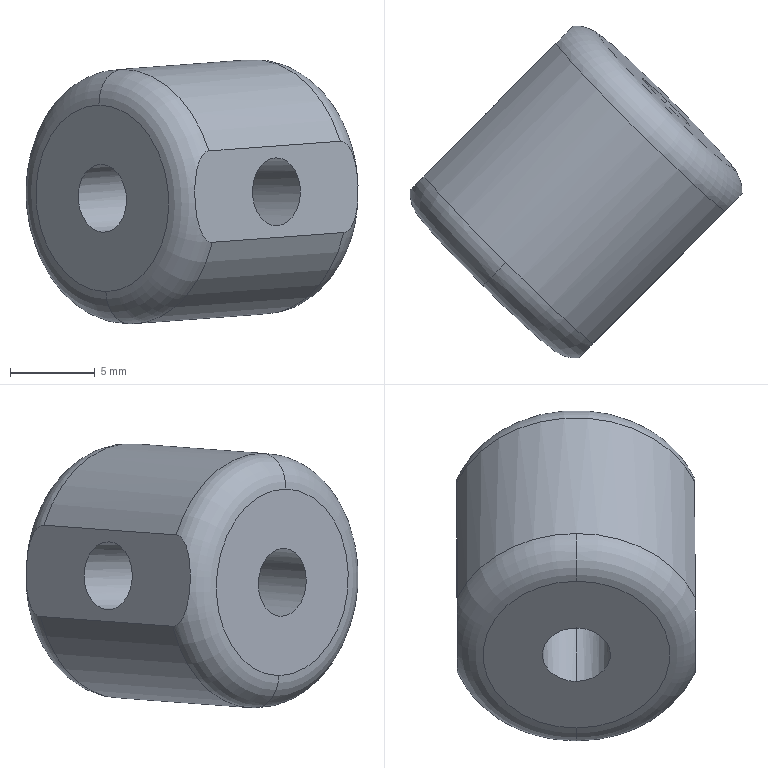Component | SolidWorks | DoubleFilmTransport-1_CrossJoint-3 | 1 solid | 19 faces | box 19.56 x 19.56 x 15.56 mm | volume 2207 mm3 | cylinder 11 | torus 4 | plane 4 | commonest cylinder face diameters 4 x8 15 x3
STEP:
#1=COLOUR_RGB('',0.7922,0.8196,0.9333);
#2=FILL_AREA_STYLE_COLOUR('',#1);
#3=FILL_AREA_STYLE('',(#2));
#4=SURFACE_STYLE_FILL_AREA(#3);
#5=SURFACE_SIDE_STYLE('',(#4));
#6=SURFACE_STYLE_USAGE(.BOTH.,#5);
#7=PRESENTATION_STYLE_ASSIGNMENT((#6));
#8=CARTESIAN_POINT('',(-15.09,3.644,-2.839));
#9=VERTEX_POINT('',#8);
#10=CARTESIAN_POINT('',(-14.783,3.339,-2.839));
#11=VERTEX_POINT('',#10);
#12=CARTESIAN_POINT('',(-14.937,3.492,-2.839));
#13=DIRECTION('',(-0.704,-0.7083,-0.05198));
#14=DIRECTION('',(-0.7092,0.705,0.));
#15=AXIS2_PLACEMENT_3D('',#12,#13,#14);
#16=CIRCLE('',#15,0.2165);
#17=EDGE_CURVE('',#9,#11,#16,.T.);
#18=ORIENTED_EDGE('',*,*,#17,.T.);
#19=CARTESIAN_POINT('',(-14.76,3.278,-2.84));
#20=VERTEX_POINT('',#19);
#21=CARTESIAN_POINT('',(-14.839,3.283,-2.843));
#22=DIRECTION('',(0.03664,0.03687,-0.9986));
#23=DIRECTION('',(0.,0.9993,0.03689));
#24=AXIS2_PLACEMENT_3D('',#21,#22,#23);
#25=CIRCLE('',#24,0.07874);
#26=EDGE_CURVE('',#11,#20,#25,.T.);
#27=ORIENTED_EDGE('',*,*,#26,.T.);
#28=CARTESIAN_POINT('',(-14.793,3.245,-2.949));
#29=VERTEX_POINT('',#28);
#30=CARTESIAN_POINT('',(-14.76,3.278,-2.84));
#31=CARTESIAN_POINT('',(-14.76,3.279,-2.851));
#32=CARTESIAN_POINT('',(-14.76,3.279,-2.862));
#33=CARTESIAN_POINT('',(-14.761,3.277,-2.883));
#34=CARTESIAN_POINT('',(-14.762,3.276,-2.893));
#35=CARTESIAN_POINT('',(-14.767,3.272,-2.914));
#36=CARTESIAN_POINT('',(-14.77,3.269,-2.924));
#37=CARTESIAN_POINT('',(-14.776,3.262,-2.937));
#38=CARTESIAN_POINT('',(-14.779,3.259,-2.941));
#39=CARTESIAN_POINT('',(-14.784,3.255,-2.945));
#40=CARTESIAN_POINT('',(-14.786,3.253,-2.947));
#41=CARTESIAN_POINT('',(-14.789,3.249,-2.948));
#42=CARTESIAN_POINT('',(-14.791,3.247,-2.949));
#43=CARTESIAN_POINT('',(-14.793,3.245,-2.949));
#44=B_SPLINE_CURVE_WITH_KNOTS('',3,(#30,#31,#32,#33,#34,#35,#36,#37,#38,#39,#40,#41,#42,#43),.UNSPECIFIED.,.F.,.F.,(4,2,2,2,2,2,4),(0.00327,0.004088,0.004906,0.005724,0.006133,0.006337,0.006542),.UNSPECIFIED.);
#45=EDGE_CURVE('',#20,#29,#44,.T.);
#46=ORIENTED_EDGE('',*,*,#45,.T.);
#47=CARTESIAN_POINT('',(-14.981,3.447,-3.138));
#48=VERTEX_POINT('',#47);
#49=CARTESIAN_POINT('',(-14.992,3.436,-2.843));
#50=DIRECTION('',(0.704,0.7083,0.05198));
#51=DIRECTION('',(-0.03664,-0.03687,0.9986));
#52=AXIS2_PLACEMENT_3D('',#49,#50,#51);
#53=CIRCLE('',#52,0.2953);
#54=EDGE_CURVE('',#29,#48,#53,.T.);
#55=ORIENTED_EDGE('',*,*,#54,.T.);
#56=CARTESIAN_POINT('',(-15.184,3.634,-2.949));
#57=VERTEX_POINT('',#56);
#58=CARTESIAN_POINT('',(-14.992,3.436,-2.843));
#59=DIRECTION('',(0.704,0.7083,0.05198));
#60=DIRECTION('',(-0.03664,-0.03687,0.9986));
#61=AXIS2_PLACEMENT_3D('',#58,#59,#60);
#62=CIRCLE('',#61,0.2953);
#63=EDGE_CURVE('',#48,#57,#62,.T.);
#64=ORIENTED_EDGE('',*,*,#63,.T.);
#65=CARTESIAN_POINT('',(-15.151,3.667,-2.84));
#66=VERTEX_POINT('',#65);
#67=CARTESIAN_POINT('',(-15.184,3.634,-2.949));
#68=CARTESIAN_POINT('',(-15.18,3.638,-2.949));
#69=CARTESIAN_POINT('',(-15.176,3.642,-2.947));
#70=CARTESIAN_POINT('',(-15.17,3.648,-2.941));
#71=CARTESIAN_POINT('',(-15.167,3.651,-2.937));
#72=CARTESIAN_POINT('',(-15.163,3.655,-2.928));
#73=CARTESIAN_POINT('',(-15.161,3.657,-2.924));
#74=CARTESIAN_POINT('',(-15.158,3.66,-2.914));
#75=CARTESIAN_POINT('',(-15.156,3.662,-2.909));
#76=CARTESIAN_POINT('',(-15.153,3.665,-2.893));
#77=CARTESIAN_POINT('',(-15.152,3.666,-2.883));
#78=CARTESIAN_POINT('',(-15.151,3.667,-2.862));
#79=CARTESIAN_POINT('',(-15.151,3.667,-2.851));
#80=CARTESIAN_POINT('',(-15.151,3.667,-2.84));
#81=B_SPLINE_CURVE_WITH_KNOTS('',3,(#67,#68,#69,#70,#71,#72,#73,#74,#75,#76,#77,#78,#79,#80),.UNSPECIFIED.,.F.,.F.,(4,2,2,2,2,2,4),(0.,0.0004087,0.0008174,0.001226,0.001635,0.002452,0.00327),.UNSPECIFIED.);
#82=EDGE_CURVE('',#57,#66,#81,.T.);
#83=ORIENTED_EDGE('',*,*,#82,.T.);
#84=CARTESIAN_POINT('',(-15.146,3.588,-2.843));
#85=DIRECTION('',(-0.03664,-0.03687,0.9986));
#86=DIRECTION('',(0.,-0.9993,-0.03689));
#87=AXIS2_PLACEMENT_3D('',#84,#85,#86);
#88=CIRCLE('',#87,0.07874);
#89=EDGE_CURVE('',#9,#66,#88,.T.);
#90=ORIENTED_EDGE('',*,*,#89,.F.);
#91=EDGE_LOOP('',(#18,#27,#46,#55,#64,#83,#90));
#92=FACE_OUTER_BOUND('',#91,.T.);
#93=CARTESIAN_POINT('',(-14.992,3.436,-2.843));
#94=DIRECTION('',(-0.704,-0.7083,-0.05198));
#95=DIRECTION('',(-0.7092,0.705,0.));
#96=AXIS2_PLACEMENT_3D('',#93,#94,#95);
#97=TOROIDAL_SURFACE('',#96,0.2165,0.07874);
#98=ADVANCED_FACE('',(#92),#97,.T.);
#99=CARTESIAN_POINT('',(-15.308,3.118,-2.571));
#100=VERTEX_POINT('',#99);
#101=CARTESIAN_POINT('',(-15.106,2.931,-2.76));
#102=VERTEX_POINT('',#101);
#103=CARTESIAN_POINT('',(-15.297,3.129,-2.866));
#104=DIRECTION('',(0.704,0.7083,0.05198));
#105=DIRECTION('',(0.03664,0.03687,-0.9986));
#106=AXIS2_PLACEMENT_3D('',#103,#104,#105);
#107=CIRCLE('',#106,0.2953);
#108=EDGE_CURVE('',#100,#102,#107,.T.);
#109=ORIENTED_EDGE('',*,*,#108,.F.);
#110=CARTESIAN_POINT('',(-15.361,3.065,-2.653));
#111=VERTEX_POINT('',#110);
#112=CARTESIAN_POINT('',(-15.305,3.121,-2.649));
#113=DIRECTION('',(0.7092,-0.705,0.));
#114=DIRECTION('',(0.705,0.7092,0.));
#115=AXIS2_PLACEMENT_3D('',#112,#113,#114);
#116=CIRCLE('',#115,0.07874);
#117=EDGE_CURVE('',#100,#111,#116,.T.);
#118=ORIENTED_EDGE('',*,*,#117,.T.);
#119=CARTESIAN_POINT('',(-15.345,3.081,-3.086));
#120=VERTEX_POINT('',#119);
#121=CARTESIAN_POINT('',(-15.353,3.073,-2.87));
#122=DIRECTION('',(0.704,0.7083,0.05198));
#123=DIRECTION('',(0.03664,0.03687,-0.9986));
#124=AXIS2_PLACEMENT_3D('',#121,#122,#123);
#125=CIRCLE('',#124,0.2165);
#126=EDGE_CURVE('',#111,#120,#125,.T.);
#127=ORIENTED_EDGE('',*,*,#126,.T.);
#128=CARTESIAN_POINT('',(-15.286,3.14,-3.16));
#129=VERTEX_POINT('',#128);
#130=CARTESIAN_POINT('',(-15.289,3.137,-3.082));
#131=DIRECTION('',(-0.7092,0.705,-0.));
#132=DIRECTION('',(-0.705,-0.7092,0.));
#133=AXIS2_PLACEMENT_3D('',#130,#131,#132);
#134=CIRCLE('',#133,0.07874);
#135=EDGE_CURVE('',#129,#120,#134,.T.);
#136=ORIENTED_EDGE('',*,*,#135,.F.);
#137=CARTESIAN_POINT('',(-15.098,2.939,-2.971));
#138=VERTEX_POINT('',#137);
#139=CARTESIAN_POINT('',(-15.297,3.129,-2.866));
#140=DIRECTION('',(-0.704,-0.7083,-0.05198));
#141=DIRECTION('',(0.03664,0.03687,-0.9986));
#142=AXIS2_PLACEMENT_3D('',#139,#140,#141);
#143=CIRCLE('',#142,0.2953);
#144=EDGE_CURVE('',#129,#138,#143,.T.);
#145=ORIENTED_EDGE('',*,*,#144,.T.);
#146=CARTESIAN_POINT('',(-15.098,2.939,-2.971));
#147=CARTESIAN_POINT('',(-15.102,2.935,-2.972));
#148=CARTESIAN_POINT('',(-15.105,2.931,-2.97));
#149=CARTESIAN_POINT('',(-15.112,2.924,-2.965));
#150=CARTESIAN_POINT('',(-15.115,2.921,-2.962));
#151=CARTESIAN_POINT('',(-15.12,2.916,-2.954));
#152=CARTESIAN_POINT('',(-15.123,2.914,-2.95));
#153=CARTESIAN_POINT('',(-15.126,2.91,-2.941));
#154=CARTESIAN_POINT('',(-15.128,2.908,-2.936));
#155=CARTESIAN_POINT('',(-15.132,2.904,-2.921));
#156=CARTESIAN_POINT('',(-15.134,2.902,-2.91));
#157=CARTESIAN_POINT('',(-15.137,2.899,-2.89));
#158=CARTESIAN_POINT('',(-15.138,2.898,-2.879));
#159=CARTESIAN_POINT('',(-15.139,2.897,-2.858));
#160=CARTESIAN_POINT('',(-15.139,2.898,-2.847));
#161=CARTESIAN_POINT('',(-15.137,2.899,-2.826));
#162=CARTESIAN_POINT('',(-15.136,2.9,-2.815));
#163=CARTESIAN_POINT('',(-15.132,2.904,-2.795));
#164=CARTESIAN_POINT('',(-15.129,2.907,-2.784));
#165=CARTESIAN_POINT('',(-15.122,2.914,-2.772));
#166=CARTESIAN_POINT('',(-15.119,2.917,-2.768));
#167=CARTESIAN_POINT('',(-15.113,2.923,-2.762));
#168=CARTESIAN_POINT('',(-15.109,2.927,-2.76));
#169=CARTESIAN_POINT('',(-15.106,2.931,-2.76));
#170=B_SPLINE_CURVE_WITH_KNOTS('',3,(#146,#147,#148,#149,#150,#151,#152,#153,#154,#155,#156,#157,#158,#159,#160,#161,#162,#163,#164,#165,#166,#167,#168,#169),.UNSPECIFIED.,.F.,.F.,(4,2,2,2,2,2,2,2,2,2,2,4),(0.,0.0004088,0.0008177,0.001227,0.001635,0.002453,0.003271,0.004088,0.004906,0.005724,0.006133,0.006542),.UNSPECIFIED.);
#171=EDGE_CURVE('',#138,#102,#170,.T.);
#172=ORIENTED_EDGE('',*,*,#171,.T.);
#173=EDGE_LOOP('',(#109,#118,#127,#136,#145,#172));
#174=FACE_OUTER_BOUND('',#173,.T.);
#175=CARTESIAN_POINT('',(-15.297,3.129,-2.866));
#176=DIRECTION('',(-0.704,-0.7083,-0.05198));
#177=DIRECTION('',(0.03664,0.03687,-0.9986));
#178=AXIS2_PLACEMENT_3D('',#175,#176,#177);
#179=TOROIDAL_SURFACE('',#178,0.2165,0.07874);
#180=ADVANCED_FACE('',(#174),#179,.T.);
#181=CARTESIAN_POINT('',(-15.337,3.48,-2.933));
#182=VERTEX_POINT('',#181);
#183=CARTESIAN_POINT('',(-15.343,3.474,-2.776));
#184=VERTEX_POINT('',#183);
#185=CARTESIAN_POINT('',(-15.34,3.477,-2.854));
#186=DIRECTION('',(-0.7092,0.705,-0.));
#187=DIRECTION('',(0.03664,0.03687,-0.9986));
#188=AXIS2_PLACEMENT_3D('',#185,#186,#187);
#189=CIRCLE('',#188,0.07874);
#190=EDGE_CURVE('',#182,#184,#189,.T.);
#191=ORIENTED_EDGE('',*,*,#190,.T.);
#192=CARTESIAN_POINT('',(-15.148,3.28,-2.776));
#193=VERTEX_POINT('',#192);
#194=CARTESIAN_POINT('',(-15.343,3.474,-2.776));
#195=DIRECTION('',(0.7092,-0.705,0.));
#196=VECTOR('',#195,39.37);
#197=LINE('',#194,#196);
#198=EDGE_CURVE('',#184,#193,#197,.T.);
#199=ORIENTED_EDGE('',*,*,#198,.T.);
#200=CARTESIAN_POINT('',(-15.142,3.285,-2.933));
#201=VERTEX_POINT('',#200);
#202=CARTESIAN_POINT('',(-15.142,3.285,-2.933));
#203=CARTESIAN_POINT('',(-15.364,3.285,-2.941));
#204=CARTESIAN_POINT('',(-15.37,3.279,-2.784));
#205=CARTESIAN_POINT('',(-15.148,3.28,-2.776));
#206=(BOUNDED_CURVE()B_SPLINE_CURVE(3,(#202,#203,#204,#205),.UNSPECIFIED.,.F.,.T.)B_SPLINE_CURVE_WITH_KNOTS((4,4),(4.712,7.854),.UNSPECIFIED.)CURVE()GEOMETRIC_REPRESENTATION_ITEM()RATIONAL_B_SPLINE_CURVE((1.,0.3333,0.3333,1.))REPRESENTATION_ITEM(''));
#207=EDGE_CURVE('',#201,#193,#206,.T.);
#208=ORIENTED_EDGE('',*,*,#207,.F.);
#209=CARTESIAN_POINT('',(-15.337,3.48,-2.933));
#210=DIRECTION('',(0.7092,-0.705,0.));
#211=VECTOR('',#210,39.37);
#212=LINE('',#209,#211);
#213=EDGE_CURVE('',#182,#201,#212,.T.);
#214=ORIENTED_EDGE('',*,*,#213,.F.);
#215=EDGE_LOOP('',(#191,#199,#208,#214));
#216=FACE_OUTER_BOUND('',#215,.T.);
#217=CARTESIAN_POINT('',(-15.34,3.477,-2.854));
#218=DIRECTION('',(0.7092,-0.705,0.));
#219=DIRECTION('',(0.03664,0.03687,-0.9986));
#220=AXIS2_PLACEMENT_3D('',#217,#218,#219);
#221=CYLINDRICAL_SURFACE('',#220,0.07874);
#222=ADVANCED_FACE('',(#216),#221,.F.);
#223=ORIENTED_EDGE('',*,*,#63,.F.);
#224=CARTESIAN_POINT('',(-15.296,3.13,-3.161));
#225=DIRECTION('',(-0.704,-0.7083,-0.05198));
#226=VECTOR('',#225,39.37);
#227=LINE('',#224,#226);
#228=EDGE_CURVE('',#48,#129,#227,.T.);
#229=ORIENTED_EDGE('',*,*,#228,.T.);
#230=CARTESIAN_POINT('',(-15.489,3.327,-2.971));
#231=VERTEX_POINT('',#230);
#232=CARTESIAN_POINT('',(-15.297,3.129,-2.866));
#233=DIRECTION('',(-0.704,-0.7083,-0.05198));
#234=DIRECTION('',(0.03664,0.03687,-0.9986));
#235=AXIS2_PLACEMENT_3D('',#232,#233,#234);
#236=CIRCLE('',#235,0.2953);
#237=EDGE_CURVE('',#231,#129,#236,.T.);
#238=ORIENTED_EDGE('',*,*,#237,.F.);
#239=CARTESIAN_POINT('',(-15.128,3.69,-2.945));
#240=DIRECTION('',(0.704,0.7083,0.05198));
#241=VECTOR('',#240,39.37);
#242=LINE('',#239,#241);
#243=EDGE_CURVE('',#231,#57,#242,.T.);
#244=ORIENTED_EDGE('',*,*,#243,.T.);
#245=EDGE_LOOP('',(#223,#229,#238,#244));
#246=FACE_OUTER_BOUND('',#245,.T.);
#247=CARTESIAN_POINT('',(-15.307,3.119,-2.866));
#248=DIRECTION('',(-0.704,-0.7083,-0.05198));
#249=DIRECTION('',(0.03664,0.03687,-0.9986));
#250=AXIS2_PLACEMENT_3D('',#247,#248,#249);
#251=CYLINDRICAL_SURFACE('',#250,0.2953);
#252=ADVANCED_FACE('',(#246),#251,.T.);
#253=CARTESIAN_POINT('',(-15.148,3.28,-2.776));
#254=CARTESIAN_POINT('',(-15.148,3.273,-2.776));
#255=CARTESIAN_POINT('',(-15.148,3.266,-2.777));
#256=CARTESIAN_POINT('',(-15.148,3.259,-2.778));
#257=CARTESIAN_POINT('',(-15.147,3.256,-2.778));
#258=CARTESIAN_POINT('',(-15.147,3.253,-2.779));
#259=CARTESIAN_POINT('',(-15.147,3.252,-2.779));
#260=CARTESIAN_POINT('',(-15.147,3.25,-2.78));
#261=CARTESIAN_POINT('',(-15.147,3.249,-2.78));
#262=CARTESIAN_POINT('',(-15.147,3.249,-2.78));
#263=CARTESIAN_POINT('',(-15.147,3.249,-2.78));
#264=CARTESIAN_POINT('',(-15.147,3.249,-2.78));
#265=CARTESIAN_POINT('',(-15.147,3.249,-2.78));
#266=CARTESIAN_POINT('',(-15.147,3.241,-2.782));
#267=CARTESIAN_POINT('',(-15.147,3.235,-2.784));
#268=CARTESIAN_POINT('',(-15.147,3.226,-2.787));
#269=CARTESIAN_POINT('',(-15.147,3.223,-2.789));
#270=CARTESIAN_POINT('',(-15.147,3.219,-2.791));
#271=CARTESIAN_POINT('',(-15.147,3.217,-2.792));
#272=CARTESIAN_POINT('',(-15.147,3.215,-2.793));
#273=CARTESIAN_POINT('',(-15.147,3.214,-2.793));
#274=CARTESIAN_POINT('',(-15.147,3.214,-2.794));
#275=CARTESIAN_POINT('',(-15.147,3.214,-2.794));
#276=CARTESIAN_POINT('',(-15.147,3.214,-2.794));
#277=CARTESIAN_POINT('',(-15.147,3.207,-2.798));
#278=CARTESIAN_POINT('',(-15.146,3.201,-2.802));
#279=CARTESIAN_POINT('',(-15.146,3.193,-2.809));
#280=CARTESIAN_POINT('',(-15.146,3.191,-2.811));
#281=CARTESIAN_POINT('',(-15.146,3.188,-2.815));
#282=CARTESIAN_POINT('',(-15.146,3.186,-2.817));
#283=CARTESIAN_POINT('',(-15.146,3.184,-2.819));
#284=CARTESIAN_POINT('',(-15.146,3.184,-2.82));
#285=CARTESIAN_POINT('',(-15.146,3.183,-2.82));
#286=CARTESIAN_POINT('',(-15.146,3.183,-2.821));
#287=CARTESIAN_POINT('',(-15.145,3.175,-2.833));
#288=CARTESIAN_POINT('',(-15.145,3.171,-2.846));
#289=CARTESIAN_POINT('',(-15.144,3.171,-2.865));
#290=CARTESIAN_POINT('',(-15.144,3.173,-2.871));
#291=CARTESIAN_POINT('',(-15.144,3.176,-2.88));
#292=CARTESIAN_POINT('',(-15.143,3.178,-2.883));
#293=CARTESIAN_POINT('',(-15.143,3.18,-2.888));
#294=CARTESIAN_POINT('',(-15.143,3.182,-2.89));
#295=CARTESIAN_POINT('',(-15.143,3.184,-2.892));
#296=CARTESIAN_POINT('',(-15.143,3.184,-2.894));
#297=CARTESIAN_POINT('',(-15.143,3.185,-2.894));
#298=CARTESIAN_POINT('',(-15.143,3.185,-2.895));
#299=CARTESIAN_POINT('',(-15.143,3.189,-2.9));
#300=CARTESIAN_POINT('',(-15.143,3.194,-2.904));
#301=CARTESIAN_POINT('',(-15.143,3.202,-2.91));
#302=CARTESIAN_POINT('',(-15.142,3.205,-2.912));
#303=CARTESIAN_POINT('',(-15.142,3.21,-2.915));
#304=CARTESIAN_POINT('',(-15.142,3.212,-2.917));
#305=CARTESIAN_POINT('',(-15.142,3.215,-2.918));
#306=CARTESIAN_POINT('',(-15.142,3.216,-2.919));
#307=CARTESIAN_POINT('',(-15.142,3.217,-2.919));
#308=CARTESIAN_POINT('',(-15.142,3.218,-2.919));
#309=CARTESIAN_POINT('',(-15.142,3.218,-2.92));
#310=CARTESIAN_POINT('',(-15.142,3.223,-2.922));
#311=CARTESIAN_POINT('',(-15.142,3.228,-2.924));
#312=CARTESIAN_POINT('',(-15.142,3.237,-2.927));
#313=CARTESIAN_POINT('',(-15.142,3.24,-2.928));
#314=CARTESIAN_POINT('',(-15.142,3.245,-2.929));
#315=CARTESIAN_POINT('',(-15.142,3.248,-2.93));
#316=CARTESIAN_POINT('',(-15.142,3.251,-2.93));
#317=CARTESIAN_POINT('',(-15.142,3.252,-2.931));
#318=CARTESIAN_POINT('',(-15.142,3.253,-2.931));
#319=CARTESIAN_POINT('',(-15.142,3.254,-2.931));
#320=CARTESIAN_POINT('',(-15.142,3.254,-2.931));
#321=CARTESIAN_POINT('',(-15.142,3.254,-2.931));
#322=CARTESIAN_POINT('',(-15.142,3.261,-2.932));
#323=CARTESIAN_POINT('',(-15.142,3.271,-2.933));
#324=CARTESIAN_POINT('',(-15.142,3.285,-2.933));
#325=B_SPLINE_CURVE_WITH_KNOTS('',3,(#253,#254,#255,#256,#257,#258,#259,#260,#261,#262,#263,#264,#265,#266,#267,#268,#269,#270,#271,#272,#273,#274,#275,#276,#277,#278,#279,#280,#281,#282,#283,#284,#285,#286,#287,#288,#289,#290,#291,#292,#293,#294,#295,#296,#297,#298,#299,#300,#301,#302,#303,#304,#305,#306,#307,#308,#309,#310,#311,#312,#313,#314,#315,#316,#317,#318,#319,#320,#321,#322,#323,#324),.UNSPECIFIED.,.F.,.F.,(4,2,2,1,1,1,1,2,2,2,2,1,1,1,2,2,2,2,1,1,2,2,2,2,2,1,1,2,2,2,2,1,1,1,2,2,2,2,1,1,1,1,2,2,4),(0.,0.0625,0.09375,0.1094,0.1172,0.1211,0.123,0.124,0.125,0.1875,0.2188,0.2344,0.2422,0.2461,0.248,0.25,0.3125,0.3438,0.3594,0.3672,0.3711,0.375,0.5,0.5625,0.5938,0.6094,0.6172,0.6211,0.625,0.6875,0.7188,0.7344,0.7422,0.7461,0.748,0.75,0.8125,0.8438,0.8594,0.8672,0.8711,0.873,0.874,0.875,1.),.UNSPECIFIED.);
#326=EDGE_CURVE('',#193,#201,#325,.T.);
#327=ORIENTED_EDGE('',*,*,#326,.F.);
#328=CARTESIAN_POINT('',(-14.952,3.085,-2.776));
#329=VERTEX_POINT('',#328);
#330=CARTESIAN_POINT('',(-15.343,3.474,-2.776));
#331=DIRECTION('',(0.7092,-0.705,0.));
#332=VECTOR('',#331,39.37);
#333=LINE('',#330,#332);
#334=EDGE_CURVE('',#193,#329,#333,.T.);
#335=ORIENTED_EDGE('',*,*,#334,.T.);
#336=CARTESIAN_POINT('',(-14.946,3.091,-2.933));
#337=VERTEX_POINT('',#336);
#338=CARTESIAN_POINT('',(-14.949,3.088,-2.854));
#339=DIRECTION('',(0.7092,-0.705,0.));
#340=DIRECTION('',(0.03664,0.03687,-0.9986));
#341=AXIS2_PLACEMENT_3D('',#338,#339,#340);
#342=CIRCLE('',#341,0.07874);
#343=EDGE_CURVE('',#329,#337,#342,.T.);
#344=ORIENTED_EDGE('',*,*,#343,.T.);
#345=CARTESIAN_POINT('',(-15.337,3.48,-2.933));
#346=DIRECTION('',(0.7092,-0.705,0.));
#347=VECTOR('',#346,39.37);
#348=LINE('',#345,#347);
#349=EDGE_CURVE('',#201,#337,#348,.T.);
#350=ORIENTED_EDGE('',*,*,#349,.F.);
#351=EDGE_LOOP('',(#327,#335,#344,#350));
#352=FACE_OUTER_BOUND('',#351,.T.);
#353=CARTESIAN_POINT('',(-15.34,3.477,-2.854));
#354=DIRECTION('',(0.7092,-0.705,0.));
#355=DIRECTION('',(0.03664,0.03687,-0.9986));
#356=AXIS2_PLACEMENT_3D('',#353,#354,#355);
#357=CYLINDRICAL_SURFACE('',#356,0.07874);
#358=ADVANCED_FACE('',(#352),#357,.F.);
#359=ORIENTED_EDGE('',*,*,#207,.T.);
#360=CARTESIAN_POINT('',(-15.356,3.07,-2.791));
#361=VERTEX_POINT('',#360);
#362=CARTESIAN_POINT('',(-15.31,3.116,-2.788));
#363=DIRECTION('',(-0.704,-0.7083,-0.05198));
#364=VECTOR('',#363,39.37);
#365=LINE('',#362,#364);
#366=EDGE_CURVE('',#193,#361,#365,.T.);
#367=ORIENTED_EDGE('',*,*,#366,.T.);
#368=CARTESIAN_POINT('',(-15.35,3.076,-2.948));
#369=VERTEX_POINT('',#368);
#370=CARTESIAN_POINT('',(-15.356,3.07,-2.791));
#371=CARTESIAN_POINT('',(-15.363,3.078,-2.791));
#372=CARTESIAN_POINT('',(-15.37,3.085,-2.793));
#373=CARTESIAN_POINT('',(-15.383,3.099,-2.801));
#374=CARTESIAN_POINT('',(-15.389,3.105,-2.807));
#375=CARTESIAN_POINT('',(-15.399,3.116,-2.821));
#376=CARTESIAN_POINT('',(-15.403,3.12,-2.83));
#377=CARTESIAN_POINT('',(-15.408,3.127,-2.849));
#378=CARTESIAN_POINT('',(-15.409,3.128,-2.859));
#379=CARTESIAN_POINT('',(-15.408,3.129,-2.88));
#380=CARTESIAN_POINT('',(-15.406,3.128,-2.89));
#381=CARTESIAN_POINT('',(-15.4,3.123,-2.909));
#382=CARTESIAN_POINT('',(-15.396,3.119,-2.918));
#383=CARTESIAN_POINT('',(-15.385,3.11,-2.933));
#384=CARTESIAN_POINT('',(-15.378,3.104,-2.938));
#385=CARTESIAN_POINT('',(-15.364,3.091,-2.946));
#386=CARTESIAN_POINT('',(-15.357,3.083,-2.948));
#387=CARTESIAN_POINT('',(-15.35,3.076,-2.948));
#388=B_SPLINE_CURVE_WITH_KNOTS('',3,(#370,#371,#372,#373,#374,#375,#376,#377,#378,#379,#380,#381,#382,#383,#384,#385,#386,#387),.UNSPECIFIED.,.F.,.F.,(4,2,2,2,2,2,2,2,4),(0.,0.125,0.25,0.375,0.5,0.625,0.75,0.875,1.),.UNSPECIFIED.);
#389=EDGE_CURVE('',#361,#369,#388,.T.);
#390=ORIENTED_EDGE('',*,*,#389,.T.);
#391=CARTESIAN_POINT('',(-15.304,3.122,-2.945));
#392=DIRECTION('',(-0.704,-0.7083,-0.05198));
#393=VECTOR('',#392,39.37);
#394=LINE('',#391,#393);
#395=EDGE_CURVE('',#201,#369,#394,.T.);
#396=ORIENTED_EDGE('',*,*,#395,.F.);
#397=EDGE_LOOP('',(#359,#367,#390,#396));
#398=FACE_OUTER_BOUND('',#397,.T.);
#399=CARTESIAN_POINT('',(-15.307,3.119,-2.866));
#400=DIRECTION('',(-0.704,-0.7083,-0.05198));
#401=DIRECTION('',(0.03664,0.03687,-0.9986));
#402=AXIS2_PLACEMENT_3D('',#399,#400,#401);
#403=CYLINDRICAL_SURFACE('',#402,0.07874);
#404=ADVANCED_FACE('',(#398),#403,.F.);
#405=CARTESIAN_POINT('',(-14.934,3.494,-2.918));
#406=VERTEX_POINT('',#405);
#407=CARTESIAN_POINT('',(-14.94,3.489,-2.76));
#408=VERTEX_POINT('',#407);
#409=CARTESIAN_POINT('',(-14.937,3.492,-2.839));
#410=DIRECTION('',(0.704,0.7083,0.05198));
#411=DIRECTION('',(0.03664,0.03687,-0.9986));
#412=AXIS2_PLACEMENT_3D('',#409,#410,#411);
#413=CIRCLE('',#412,0.07874);
#414=EDGE_CURVE('',#406,#408,#413,.T.);
#415=ORIENTED_EDGE('',*,*,#414,.T.);
#416=CARTESIAN_POINT('',(-15.31,3.116,-2.788));
#417=DIRECTION('',(-0.704,-0.7083,-0.05198));
#418=VECTOR('',#417,39.37);
#419=LINE('',#416,#418);
#420=EDGE_CURVE('',#408,#193,#419,.T.);
#421=ORIENTED_EDGE('',*,*,#420,.T.);
#422=CARTESIAN_POINT('',(-15.148,3.28,-2.776));
#423=CARTESIAN_POINT('',(-15.148,3.502,-2.768));
#424=CARTESIAN_POINT('',(-15.143,3.508,-2.925));
#425=CARTESIAN_POINT('',(-15.142,3.285,-2.933));
#426=(BOUNDED_CURVE()B_SPLINE_CURVE(3,(#422,#423,#424,#425),.UNSPECIFIED.,.F.,.T.)B_SPLINE_CURVE_WITH_KNOTS((4,4),(1.571,4.712),.UNSPECIFIED.)CURVE()GEOMETRIC_REPRESENTATION_ITEM()RATIONAL_B_SPLINE_CURVE((1.,0.3333,0.3333,1.))REPRESENTATION_ITEM(''));
#427=EDGE_CURVE('',#193,#201,#426,.T.);
#428=ORIENTED_EDGE('',*,*,#427,.T.);
#429=CARTESIAN_POINT('',(-15.304,3.122,-2.945));
#430=DIRECTION('',(-0.704,-0.7083,-0.05198));
#431=VECTOR('',#430,39.37);
#432=LINE('',#429,#431);
#433=EDGE_CURVE('',#406,#201,#432,.T.);
#434=ORIENTED_EDGE('',*,*,#433,.F.);
#435=EDGE_LOOP('',(#415,#421,#428,#434));
#436=FACE_OUTER_BOUND('',#435,.T.);
#437=CARTESIAN_POINT('',(-15.307,3.119,-2.866));
#438=DIRECTION('',(-0.704,-0.7083,-0.05198));
#439=DIRECTION('',(0.03664,0.03687,-0.9986));
#440=AXIS2_PLACEMENT_3D('',#437,#438,#439);
#441=CYLINDRICAL_SURFACE('',#440,0.07874);
#442=ADVANCED_FACE('',(#436),#441,.F.);
#443=CARTESIAN_POINT('',(-14.801,3.238,-2.737));
#444=VERTEX_POINT('',#443);
#445=CARTESIAN_POINT('',(-15.192,3.626,-2.737));
#446=VERTEX_POINT('',#445);
#447=CARTESIAN_POINT('',(-14.992,3.436,-2.843));
#448=DIRECTION('',(-0.704,-0.7083,-0.05198));
#449=DIRECTION('',(0.03664,0.03687,-0.9986));
#450=AXIS2_PLACEMENT_3D('',#447,#448,#449);
#451=CIRCLE('',#450,0.2953);
#452=EDGE_CURVE('',#444,#446,#451,.T.);
#453=ORIENTED_EDGE('',*,*,#452,.T.);
#454=CARTESIAN_POINT('',(-15.497,3.319,-2.76));
#455=VERTEX_POINT('',#454);
#456=CARTESIAN_POINT('',(-15.506,3.309,-2.76));
#457=DIRECTION('',(-0.704,-0.7083,-0.05198));
#458=VECTOR('',#457,39.37);
#459=LINE('',#456,#458);
#460=EDGE_CURVE('',#446,#455,#459,.T.);
#461=ORIENTED_EDGE('',*,*,#460,.T.);
#462=CARTESIAN_POINT('',(-15.297,3.129,-2.866));
#463=DIRECTION('',(0.704,0.7083,0.05198));
#464=DIRECTION('',(0.03664,0.03687,-0.9986));
#465=AXIS2_PLACEMENT_3D('',#462,#463,#464);
#466=CIRCLE('',#465,0.2953);
#467=EDGE_CURVE('',#455,#100,#466,.T.);
#468=ORIENTED_EDGE('',*,*,#467,.T.);
#469=ORIENTED_EDGE('',*,*,#108,.T.);
#470=CARTESIAN_POINT('',(-15.115,2.921,-2.76));
#471=DIRECTION('',(0.704,0.7083,0.05198));
#472=VECTOR('',#471,39.37);
#473=LINE('',#470,#472);
#474=EDGE_CURVE('',#102,#444,#473,.T.);
#475=ORIENTED_EDGE('',*,*,#474,.T.);
#476=EDGE_LOOP('',(#453,#461,#468,#469,#475));
#477=FACE_OUTER_BOUND('',#476,.T.);
#478=CARTESIAN_POINT('',(-15.307,3.119,-2.866));
#479=DIRECTION('',(-0.704,-0.7083,-0.05198));
#480=DIRECTION('',(0.03664,0.03687,-0.9986));
#481=AXIS2_PLACEMENT_3D('',#478,#479,#480);
#482=CYLINDRICAL_SURFACE('',#481,0.2953);
#483=ADVANCED_FACE('',(#477),#482,.T.);
#484=ORIENTED_EDGE('',*,*,#190,.F.);
#485=CARTESIAN_POINT('',(-15.34,3.477,-2.854));
#486=DIRECTION('',(-0.7092,0.705,-0.));
#487=DIRECTION('',(0.03664,0.03687,-0.9986));
#488=AXIS2_PLACEMENT_3D('',#485,#486,#487);
#489=CIRCLE('',#488,0.07874);
#490=EDGE_CURVE('',#184,#182,#489,.T.);
#491=ORIENTED_EDGE('',*,*,#490,.F.);
#492=EDGE_LOOP('',(#484,#491));
#493=FACE_BOUND('',#492,.T.);
#494=CARTESIAN_POINT('',(-15.497,3.319,-2.76));
#495=CARTESIAN_POINT('',(-15.5,3.316,-2.76));
#496=CARTESIAN_POINT('',(-15.504,3.312,-2.762));
#497=CARTESIAN_POINT('',(-15.51,3.305,-2.768));
#498=CARTESIAN_POINT('',(-15.513,3.303,-2.772));
#499=CARTESIAN_POINT('',(-15.518,3.298,-2.78));
#500=CARTESIAN_POINT('',(-15.52,3.296,-2.785));
#501=CARTESIAN_POINT('',(-15.523,3.293,-2.795));
#502=CARTESIAN_POINT('',(-15.524,3.292,-2.8));
#503=CARTESIAN_POINT('',(-15.527,3.289,-2.815));
#504=CARTESIAN_POINT('',(-15.528,3.287,-2.826));
#505=CARTESIAN_POINT('',(-15.53,3.286,-2.847));
#506=CARTESIAN_POINT('',(-15.53,3.286,-2.858));
#507=CARTESIAN_POINT('',(-15.529,3.287,-2.879));
#508=CARTESIAN_POINT('',(-15.528,3.288,-2.89));
#509=CARTESIAN_POINT('',(-15.525,3.291,-2.91));
#510=CARTESIAN_POINT('',(-15.523,3.293,-2.921));
#511=CARTESIAN_POINT('',(-15.518,3.298,-2.941));
#512=CARTESIAN_POINT('',(-15.514,3.302,-2.95));
#513=CARTESIAN_POINT('',(-15.506,3.31,-2.962));
#514=CARTESIAN_POINT('',(-15.503,3.313,-2.966));
#515=CARTESIAN_POINT('',(-15.496,3.32,-2.97));
#516=CARTESIAN_POINT('',(-15.493,3.323,-2.972));
#517=CARTESIAN_POINT('',(-15.489,3.327,-2.971));
#518=B_SPLINE_CURVE_WITH_KNOTS('',3,(#494,#495,#496,#497,#498,#499,#500,#501,#502,#503,#504,#505,#506,#507,#508,#509,#510,#511,#512,#513,#514,#515,#516,#517),.UNSPECIFIED.,.F.,.F.,(4,2,2,2,2,2,2,2,2,2,2,4),(0.,0.0004088,0.0008177,0.001227,0.001635,0.002453,0.003271,0.004088,0.004906,0.005724,0.006133,0.006542),.UNSPECIFIED.);
#519=EDGE_CURVE('',#455,#231,#518,.T.);
#520=ORIENTED_EDGE('',*,*,#519,.F.);
#521=ORIENTED_EDGE('',*,*,#460,.F.);
#522=CARTESIAN_POINT('',(-15.151,3.667,-2.84));
#523=CARTESIAN_POINT('',(-15.152,3.667,-2.83));
#524=CARTESIAN_POINT('',(-15.152,3.666,-2.819));
#525=CARTESIAN_POINT('',(-15.155,3.663,-2.798));
#526=CARTESIAN_POINT('',(-15.157,3.661,-2.788));
#527=CARTESIAN_POINT('',(-15.163,3.655,-2.768));
#528=CARTESIAN_POINT('',(-15.167,3.651,-2.758));
#529=CARTESIAN_POINT('',(-15.174,3.644,-2.747));
#530=CARTESIAN_POINT('',(-15.177,3.641,-2.743));
#531=CARTESIAN_POINT('',(-15.182,3.635,-2.739));
#532=CARTESIAN_POINT('',(-15.184,3.634,-2.739));
#533=CARTESIAN_POINT('',(-15.188,3.63,-2.737));
#534=CARTESIAN_POINT('',(-15.19,3.628,-2.737));
#535=CARTESIAN_POINT('',(-15.192,3.626,-2.737));
#536=B_SPLINE_CURVE_WITH_KNOTS('',3,(#522,#523,#524,#525,#526,#527,#528,#529,#530,#531,#532,#533,#534,#535),.UNSPECIFIED.,.F.,.F.,(4,2,2,2,2,2,4),(0.00327,0.004088,0.004906,0.005724,0.006133,0.006337,0.006542),.UNSPECIFIED.);
#537=EDGE_CURVE('',#66,#446,#536,.T.);
#538=ORIENTED_EDGE('',*,*,#537,.F.);
#539=ORIENTED_EDGE('',*,*,#82,.F.);
#540=ORIENTED_EDGE('',*,*,#243,.F.);
#541=EDGE_LOOP('',(#520,#521,#538,#539,#540));
#542=FACE_OUTER_BOUND('',#541,.T.);
#543=CARTESIAN_POINT('',(-15.128,3.69,-2.945));
#544=DIRECTION('',(0.7092,-0.705,0.));
#545=DIRECTION('',(0.03664,0.03687,-0.9986));
#546=AXIS2_PLACEMENT_3D('',#543,#544,#545);
#547=PLANE('',#546);
#548=ADVANCED_FACE('',(#493,#542),#547,.F.);
#549=ORIENTED_EDGE('',*,*,#26,.F.);
#550=CARTESIAN_POINT('',(-14.937,3.492,-2.839));
#551=DIRECTION('',(-0.704,-0.7083,-0.05198));
#552=DIRECTION('',(-0.7092,0.705,0.));
#553=AXIS2_PLACEMENT_3D('',#550,#551,#552);
#554=CIRCLE('',#553,0.2165);
#555=EDGE_CURVE('',#11,#9,#554,.T.);
#556=ORIENTED_EDGE('',*,*,#555,.T.);
#557=ORIENTED_EDGE('',*,*,#89,.T.);
#558=ORIENTED_EDGE('',*,*,#537,.T.);
#559=ORIENTED_EDGE('',*,*,#452,.F.);
#560=CARTESIAN_POINT('',(-14.801,3.238,-2.737));
#561=CARTESIAN_POINT('',(-14.797,3.241,-2.737));
#562=CARTESIAN_POINT('',(-14.793,3.245,-2.738));
#563=CARTESIAN_POINT('',(-14.786,3.252,-2.743));
#564=CARTESIAN_POINT('',(-14.783,3.255,-2.747));
#565=CARTESIAN_POINT('',(-14.778,3.26,-2.754));
#566=CARTESIAN_POINT('',(-14.776,3.263,-2.759));
#567=CARTESIAN_POINT('',(-14.772,3.266,-2.768));
#568=CARTESIAN_POINT('',(-14.771,3.268,-2.773));
#569=CARTESIAN_POINT('',(-14.766,3.272,-2.788));
#570=CARTESIAN_POINT('',(-14.764,3.274,-2.798));
#571=CARTESIAN_POINT('',(-14.761,3.277,-2.819));
#572=CARTESIAN_POINT('',(-14.761,3.278,-2.83));
#573=CARTESIAN_POINT('',(-14.76,3.278,-2.84));
#574=B_SPLINE_CURVE_WITH_KNOTS('',3,(#560,#561,#562,#563,#564,#565,#566,#567,#568,#569,#570,#571,#572,#573),.UNSPECIFIED.,.F.,.F.,(4,2,2,2,2,2,4),(0.,0.0004087,0.0008174,0.001226,0.001635,0.002452,0.00327),.UNSPECIFIED.);
#575=EDGE_CURVE('',#444,#20,#574,.T.);
#576=ORIENTED_EDGE('',*,*,#575,.T.);
#577=EDGE_LOOP('',(#549,#556,#557,#558,#559,#576));
#578=FACE_OUTER_BOUND('',#577,.T.);
#579=CARTESIAN_POINT('',(-14.992,3.436,-2.843));
#580=DIRECTION('',(-0.704,-0.7083,-0.05198));
#581=DIRECTION('',(-0.7092,0.705,0.));
#582=AXIS2_PLACEMENT_3D('',#579,#580,#581);
#583=TOROIDAL_SURFACE('',#582,0.2165,0.07874);
#584=ADVANCED_FACE('',(#578),#583,.T.);
#585=CARTESIAN_POINT('',(-14.949,3.088,-2.854));
#586=DIRECTION('',(0.7092,-0.705,0.));
#587=DIRECTION('',(0.03664,0.03687,-0.9986));
#588=AXIS2_PLACEMENT_3D('',#585,#586,#587);
#589=CIRCLE('',#588,0.07874);
#590=EDGE_CURVE('',#337,#329,#589,.T.);
#591=ORIENTED_EDGE('',*,*,#590,.F.);
#592=ORIENTED_EDGE('',*,*,#343,.F.);
#593=EDGE_LOOP('',(#591,#592));
#594=FACE_BOUND('',#593,.T.);
#595=ORIENTED_EDGE('',*,*,#171,.F.);
#596=CARTESIAN_POINT('',(-14.738,3.301,-2.945));
#597=DIRECTION('',(-0.704,-0.7083,-0.05198));
#598=VECTOR('',#597,39.37);
#599=LINE('',#596,#598);
#600=EDGE_CURVE('',#29,#138,#599,.T.);
#601=ORIENTED_EDGE('',*,*,#600,.F.);
#602=ORIENTED_EDGE('',*,*,#45,.F.);
#603=ORIENTED_EDGE('',*,*,#575,.F.);
#604=ORIENTED_EDGE('',*,*,#474,.F.);
#605=EDGE_LOOP('',(#595,#601,#602,#603,#604));
#606=FACE_OUTER_BOUND('',#605,.T.);
#607=CARTESIAN_POINT('',(-14.745,3.293,-2.733));
#608=DIRECTION('',(-0.7092,0.705,-0.));
#609=DIRECTION('',(-0.03664,-0.03687,0.9986));
#610=AXIS2_PLACEMENT_3D('',#607,#608,#609);
#611=PLANE('',#610);
#612=ADVANCED_FACE('',(#594,#606),#611,.F.);
#613=ORIENTED_EDGE('',*,*,#117,.F.);
#614=ORIENTED_EDGE('',*,*,#467,.F.);
#615=ORIENTED_EDGE('',*,*,#519,.T.);
#616=ORIENTED_EDGE('',*,*,#237,.T.);
#617=ORIENTED_EDGE('',*,*,#135,.T.);
#618=CARTESIAN_POINT('',(-15.353,3.073,-2.87));
#619=DIRECTION('',(0.704,0.7083,0.05198));
#620=DIRECTION('',(0.03664,0.03687,-0.9986));
#621=AXIS2_PLACEMENT_3D('',#618,#619,#620);
#622=CIRCLE('',#621,0.2165);
#623=EDGE_CURVE('',#120,#111,#622,.T.);
#624=ORIENTED_EDGE('',*,*,#623,.T.);
#625=EDGE_LOOP('',(#613,#614,#615,#616,#617,#624));
#626=FACE_OUTER_BOUND('',#625,.T.);
#627=CARTESIAN_POINT('',(-15.297,3.129,-2.866));
#628=DIRECTION('',(-0.704,-0.7083,-0.05198));
#629=DIRECTION('',(0.03664,0.03687,-0.9986));
#630=AXIS2_PLACEMENT_3D('',#627,#628,#629);
#631=TOROIDAL_SURFACE('',#630,0.2165,0.07874);
#632=ADVANCED_FACE('',(#626),#631,.T.);
#633=ORIENTED_EDGE('',*,*,#198,.F.);
#634=ORIENTED_EDGE('',*,*,#490,.T.);
#635=ORIENTED_EDGE('',*,*,#213,.T.);
#636=ORIENTED_EDGE('',*,*,#427,.F.);
#637=EDGE_LOOP('',(#633,#634,#635,#636));
#638=FACE_OUTER_BOUND('',#637,.T.);
#639=CARTESIAN_POINT('',(-15.34,3.477,-2.854));
#640=DIRECTION('',(0.7092,-0.705,0.));
#641=DIRECTION('',(0.03664,0.03687,-0.9986));
#642=AXIS2_PLACEMENT_3D('',#639,#640,#641);
#643=CYLINDRICAL_SURFACE('',#642,0.07874);
#644=ADVANCED_FACE('',(#638),#643,.F.);
#645=ORIENTED_EDGE('',*,*,#228,.F.);
#646=ORIENTED_EDGE('',*,*,#54,.F.);
#647=ORIENTED_EDGE('',*,*,#600,.T.);
#648=ORIENTED_EDGE('',*,*,#144,.F.);
#649=EDGE_LOOP('',(#645,#646,#647,#648));
#650=FACE_OUTER_BOUND('',#649,.T.);
#651=CARTESIAN_POINT('',(-15.307,3.119,-2.866));
#652=DIRECTION('',(-0.704,-0.7083,-0.05198));
#653=DIRECTION('',(0.03664,0.03687,-0.9986));
#654=AXIS2_PLACEMENT_3D('',#651,#652,#653);
#655=CYLINDRICAL_SURFACE('',#654,0.2953);
#656=ADVANCED_FACE('',(#650),#655,.T.);
#657=ORIENTED_EDGE('',*,*,#17,.F.);
#658=ORIENTED_EDGE('',*,*,#555,.F.);
#659=EDGE_LOOP('',(#657,#658));
#660=FACE_OUTER_BOUND('',#659,.T.);
#661=ORIENTED_EDGE('',*,*,#414,.F.);
#662=CARTESIAN_POINT('',(-14.937,3.492,-2.839));
#663=DIRECTION('',(0.704,0.7083,0.05198));
#664=DIRECTION('',(0.03664,0.03687,-0.9986));
#665=AXIS2_PLACEMENT_3D('',#662,#663,#664);
#666=CIRCLE('',#665,0.07874);
#667=EDGE_CURVE('',#408,#406,#666,.T.);
#668=ORIENTED_EDGE('',*,*,#667,.F.);
#669=EDGE_LOOP('',(#661,#668));
#670=FACE_BOUND('',#669,.T.);
#671=CARTESIAN_POINT('',(-14.881,3.436,-2.839));
#672=DIRECTION('',(-0.704,-0.7083,-0.05198));
#673=DIRECTION('',(0.03664,0.03687,-0.9986));
#674=AXIS2_PLACEMENT_3D('',#671,#672,#673);
#675=PLANE('',#674);
#676=ADVANCED_FACE('',(#660,#670),#675,.F.);
#677=ORIENTED_EDGE('',*,*,#334,.F.);
#678=CARTESIAN_POINT('',(-15.142,3.285,-2.933));
#679=CARTESIAN_POINT('',(-14.919,3.286,-2.925));
#680=CARTESIAN_POINT('',(-14.925,3.28,-2.768));
#681=CARTESIAN_POINT('',(-15.148,3.28,-2.776));
#682=(BOUNDED_CURVE()B_SPLINE_CURVE(3,(#678,#679,#680,#681),.UNSPECIFIED.,.F.,.F.)B_SPLINE_CURVE_WITH_KNOTS((4,4),(1.571,4.712),.UNSPECIFIED.)CURVE()GEOMETRIC_REPRESENTATION_ITEM()RATIONAL_B_SPLINE_CURVE((1.,0.3333,0.3333,1.))REPRESENTATION_ITEM(''));
#683=EDGE_CURVE('',#201,#193,#682,.T.);
#684=ORIENTED_EDGE('',*,*,#683,.F.);
#685=ORIENTED_EDGE('',*,*,#349,.T.);
#686=ORIENTED_EDGE('',*,*,#590,.T.);
#687=EDGE_LOOP('',(#677,#684,#685,#686));
#688=FACE_OUTER_BOUND('',#687,.T.);
#689=CARTESIAN_POINT('',(-15.34,3.477,-2.854));
#690=DIRECTION('',(0.7092,-0.705,0.));
#691=DIRECTION('',(0.03664,0.03687,-0.9986));
#692=AXIS2_PLACEMENT_3D('',#689,#690,#691);
#693=CYLINDRICAL_SURFACE('',#692,0.07874);
#694=ADVANCED_FACE('',(#688),#693,.F.);
#695=ORIENTED_EDGE('',*,*,#389,.F.);
#696=CARTESIAN_POINT('',(-15.35,3.076,-2.948));
#697=CARTESIAN_POINT('',(-15.342,3.069,-2.948));
#698=CARTESIAN_POINT('',(-15.335,3.062,-2.946));
#699=CARTESIAN_POINT('',(-15.322,3.048,-2.938));
#700=CARTESIAN_POINT('',(-15.316,3.041,-2.933));
#701=CARTESIAN_POINT('',(-15.306,3.031,-2.918));
#702=CARTESIAN_POINT('',(-15.302,3.026,-2.909));
#703=CARTESIAN_POINT('',(-15.297,3.02,-2.89));
#704=CARTESIAN_POINT('',(-15.296,3.018,-2.88));
#705=CARTESIAN_POINT('',(-15.297,3.017,-2.859));
#706=CARTESIAN_POINT('',(-15.299,3.018,-2.849));
#707=CARTESIAN_POINT('',(-15.305,3.023,-2.83));
#708=CARTESIAN_POINT('',(-15.31,3.027,-2.821));
#709=CARTESIAN_POINT('',(-15.321,3.037,-2.807));
#710=CARTESIAN_POINT('',(-15.327,3.043,-2.801));
#711=CARTESIAN_POINT('',(-15.341,3.056,-2.793));
#712=CARTESIAN_POINT('',(-15.348,3.063,-2.791));
#713=CARTESIAN_POINT('',(-15.356,3.07,-2.791));
#714=B_SPLINE_CURVE_WITH_KNOTS('',3,(#696,#697,#698,#699,#700,#701,#702,#703,#704,#705,#706,#707,#708,#709,#710,#711,#712,#713),.UNSPECIFIED.,.F.,.F.,(4,2,2,2,2,2,2,2,4),(0.,0.125,0.25,0.375,0.5,0.625,0.75,0.875,1.),.UNSPECIFIED.);
#715=EDGE_CURVE('',#369,#361,#714,.T.);
#716=ORIENTED_EDGE('',*,*,#715,.F.);
#717=EDGE_LOOP('',(#695,#716));
#718=FACE_BOUND('',#717,.T.);
#719=ORIENTED_EDGE('',*,*,#623,.F.);
#720=ORIENTED_EDGE('',*,*,#126,.F.);
#721=EDGE_LOOP('',(#719,#720));
#722=FACE_OUTER_BOUND('',#721,.T.);
#723=CARTESIAN_POINT('',(-15.199,2.921,-2.87));
#724=DIRECTION('',(0.704,0.7083,0.05198));
#725=DIRECTION('',(-0.03664,-0.03687,0.9986));
#726=AXIS2_PLACEMENT_3D('',#723,#724,#725);
#727=PLANE('',#726);
#728=ADVANCED_FACE('',(#718,#722),#727,.F.);
#729=ORIENTED_EDGE('',*,*,#366,.F.);
#730=ORIENTED_EDGE('',*,*,#326,.T.);
#731=ORIENTED_EDGE('',*,*,#395,.T.);
#732=ORIENTED_EDGE('',*,*,#715,.T.);
#733=EDGE_LOOP('',(#729,#730,#731,#732));
#734=FACE_OUTER_BOUND('',#733,.T.);
#735=CARTESIAN_POINT('',(-15.307,3.119,-2.866));
#736=DIRECTION('',(-0.704,-0.7083,-0.05198));
#737=DIRECTION('',(0.03664,0.03687,-0.9986));
#738=AXIS2_PLACEMENT_3D('',#735,#736,#737);
#739=CYLINDRICAL_SURFACE('',#738,0.07874);
#740=ADVANCED_FACE('',(#734),#739,.F.);
#741=ORIENTED_EDGE('',*,*,#420,.F.);
#742=ORIENTED_EDGE('',*,*,#667,.T.);
#743=ORIENTED_EDGE('',*,*,#433,.T.);
#744=ORIENTED_EDGE('',*,*,#683,.T.);
#745=EDGE_LOOP('',(#741,#742,#743,#744));
#746=FACE_OUTER_BOUND('',#745,.T.);
#747=CARTESIAN_POINT('',(-15.307,3.119,-2.866));
#748=DIRECTION('',(-0.704,-0.7083,-0.05198));
#749=DIRECTION('',(0.03664,0.03687,-0.9986));
#750=AXIS2_PLACEMENT_3D('',#747,#748,#749);
#751=CYLINDRICAL_SURFACE('',#750,0.07874);
#752=ADVANCED_FACE('',(#746),#751,.F.);
#753=CLOSED_SHELL('',(#98,#180,#222,#252,#358,#404,#442,#483,#548,#584,#612,#632,#644,#656,#676,#694,#728,#740,#752));
#754=MANIFOLD_SOLID_BREP('',#753);
#755=STYLED_ITEM('',(#7),#754);
#756=PRESENTATION_LAYER_ASSIGNMENT('','',(#755));
#757=CARTESIAN_POINT('',(0.,0.,0.));
#758=DIRECTION('',(0.,0.,1.));
#759=DIRECTION('',(1.,0.,0.));
#760=AXIS2_PLACEMENT_3D('',#757,#758,#759);
#761=(LENGTH_UNIT()NAMED_UNIT(*)SI_UNIT($,.METRE.));
#762=LENGTH_MEASURE_WITH_UNIT(LENGTH_MEASURE(0.0254),#761);
#763=DIMENSIONAL_EXPONENTS(1.,0.,0.,0.,0.,0.,0.);
#764=(CONVERSION_BASED_UNIT('',#762)LENGTH_UNIT()NAMED_UNIT(#763));
#765=UNCERTAINTY_MEASURE_WITH_UNIT(LENGTH_MEASURE(0.00001),#764,'','');
#766=(NAMED_UNIT(*)PLANE_ANGLE_UNIT()SI_UNIT($,.RADIAN.));
#767=(NAMED_UNIT(*)SI_UNIT($,.STERADIAN.)SOLID_ANGLE_UNIT());
#768=(GEOMETRIC_REPRESENTATION_CONTEXT(3)GLOBAL_UNCERTAINTY_ASSIGNED_CONTEXT((#765))GLOBAL_UNIT_ASSIGNED_CONTEXT((#764,#766,#767))REPRESENTATION_CONTEXT('',''));
#769=ADVANCED_BREP_SHAPE_REPRESENTATION('',(#754,#760),#768);
#770=(LENGTH_UNIT()NAMED_UNIT(*)SI_UNIT($,.METRE.));
#771=LENGTH_MEASURE_WITH_UNIT(LENGTH_MEASURE(0.0254),#770);
#772=DIMENSIONAL_EXPONENTS(1.,0.,0.,0.,0.,0.,0.);
#773=(CONVERSION_BASED_UNIT('',#771)LENGTH_UNIT()NAMED_UNIT(#772));
#774=UNCERTAINTY_MEASURE_WITH_UNIT(LENGTH_MEASURE(0.00001),#773,'','');
#775=(NAMED_UNIT(*)PLANE_ANGLE_UNIT()SI_UNIT($,.RADIAN.));
#776=(NAMED_UNIT(*)SI_UNIT($,.STERADIAN.)SOLID_ANGLE_UNIT());
#777=(GEOMETRIC_REPRESENTATION_CONTEXT(3)GLOBAL_UNCERTAINTY_ASSIGNED_CONTEXT((#774))GLOBAL_UNIT_ASSIGNED_CONTEXT((#773,#775,#776))REPRESENTATION_CONTEXT('',''));
#778=MECHANICAL_DESIGN_GEOMETRIC_PRESENTATION_REPRESENTATION('',(#755),#777);